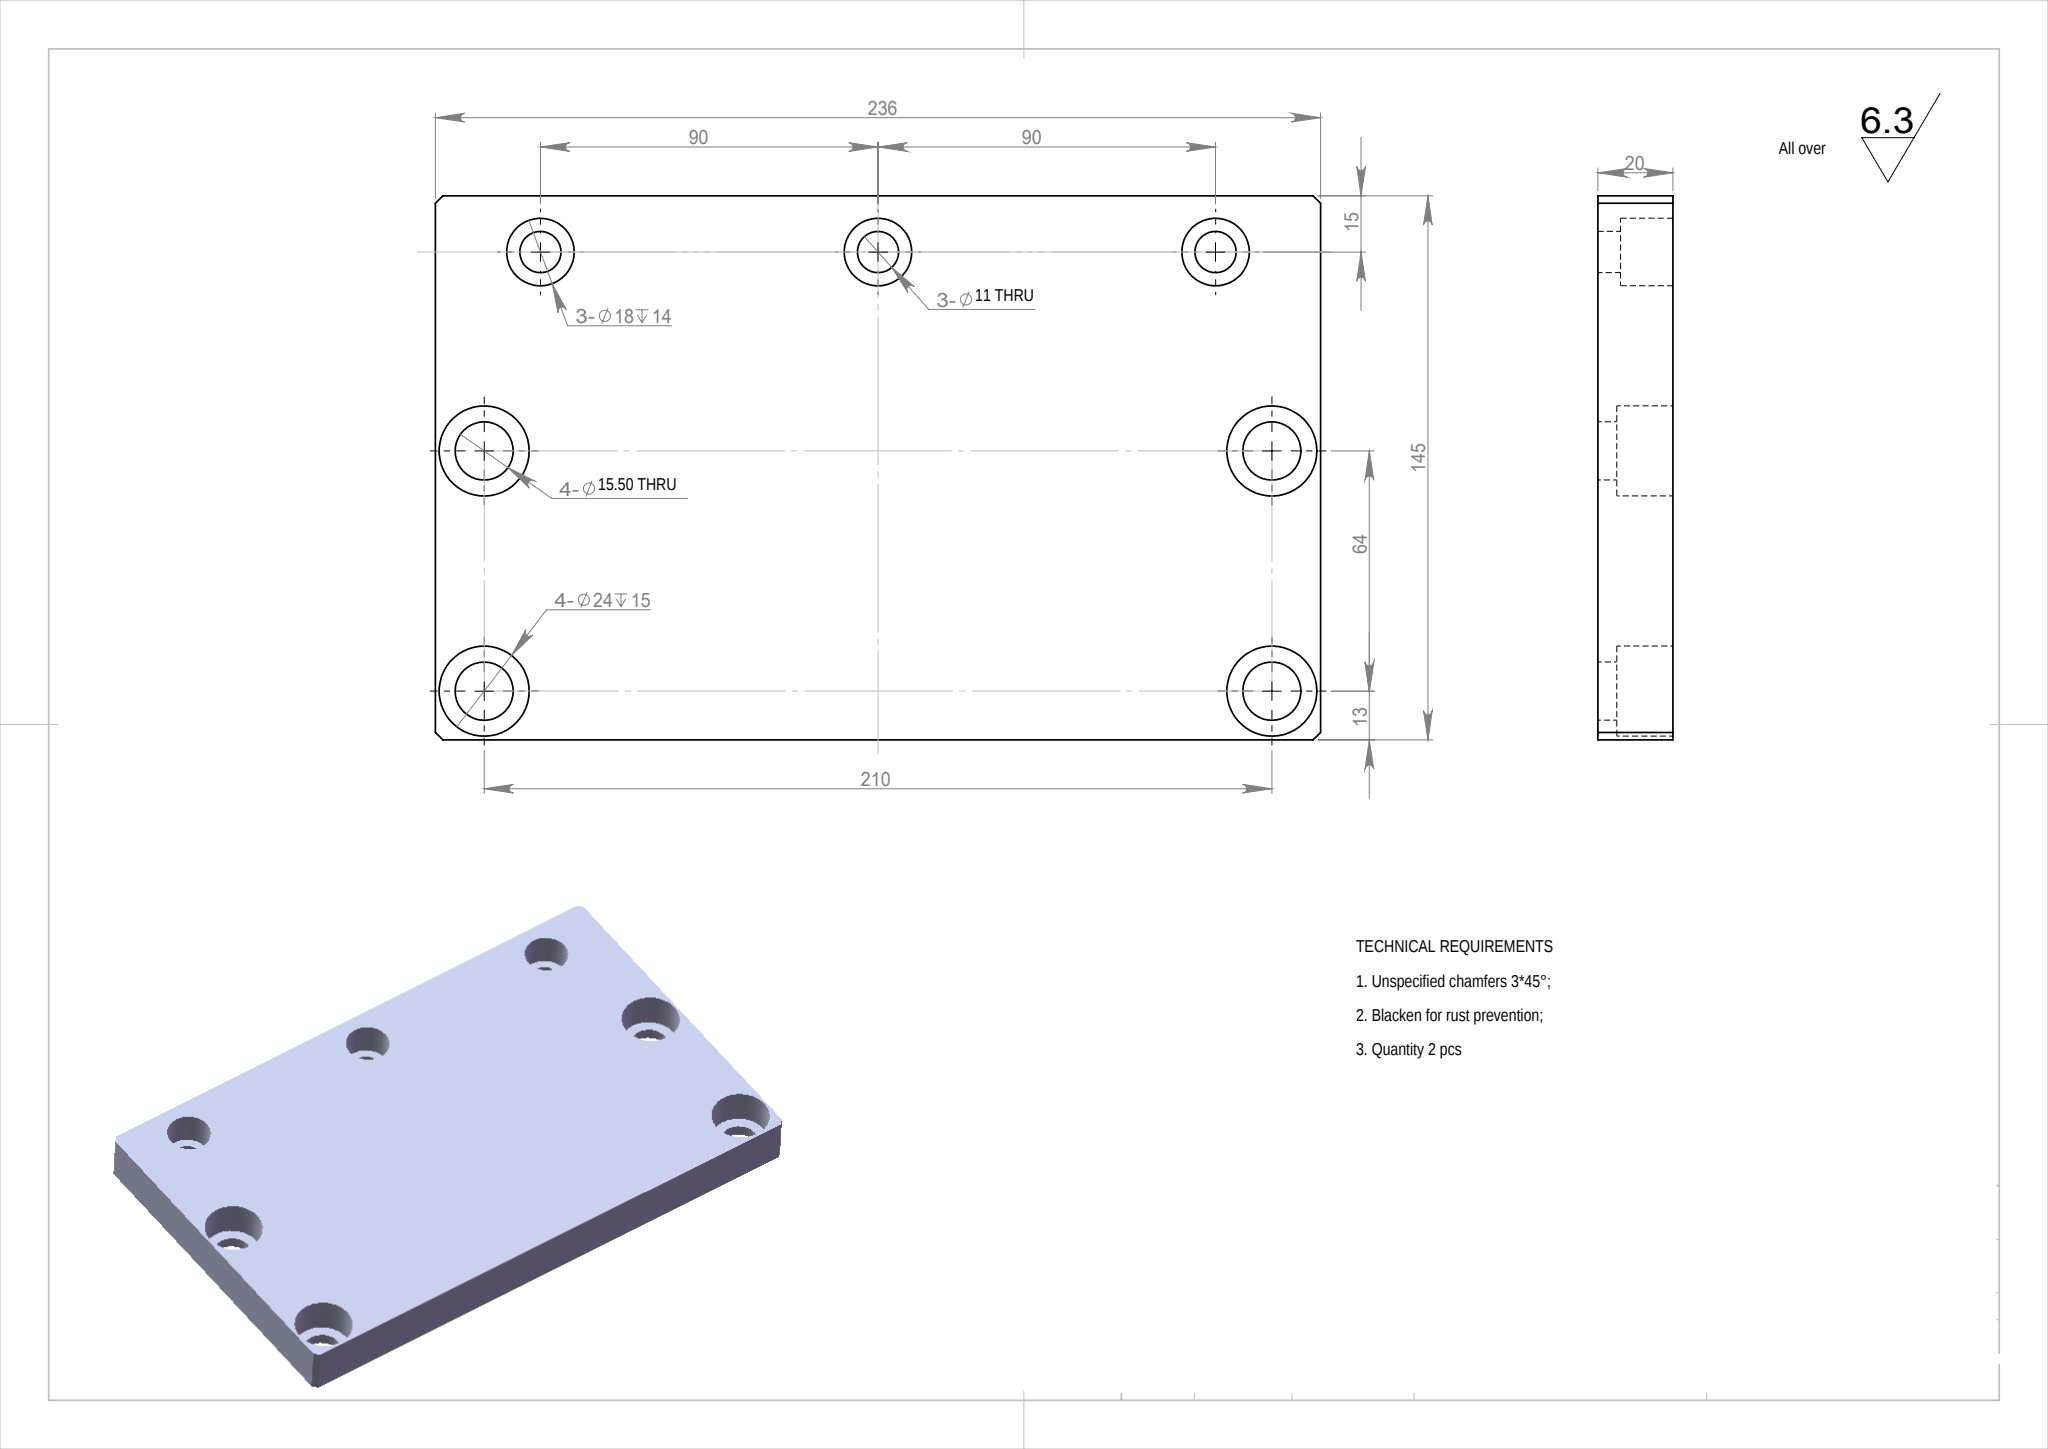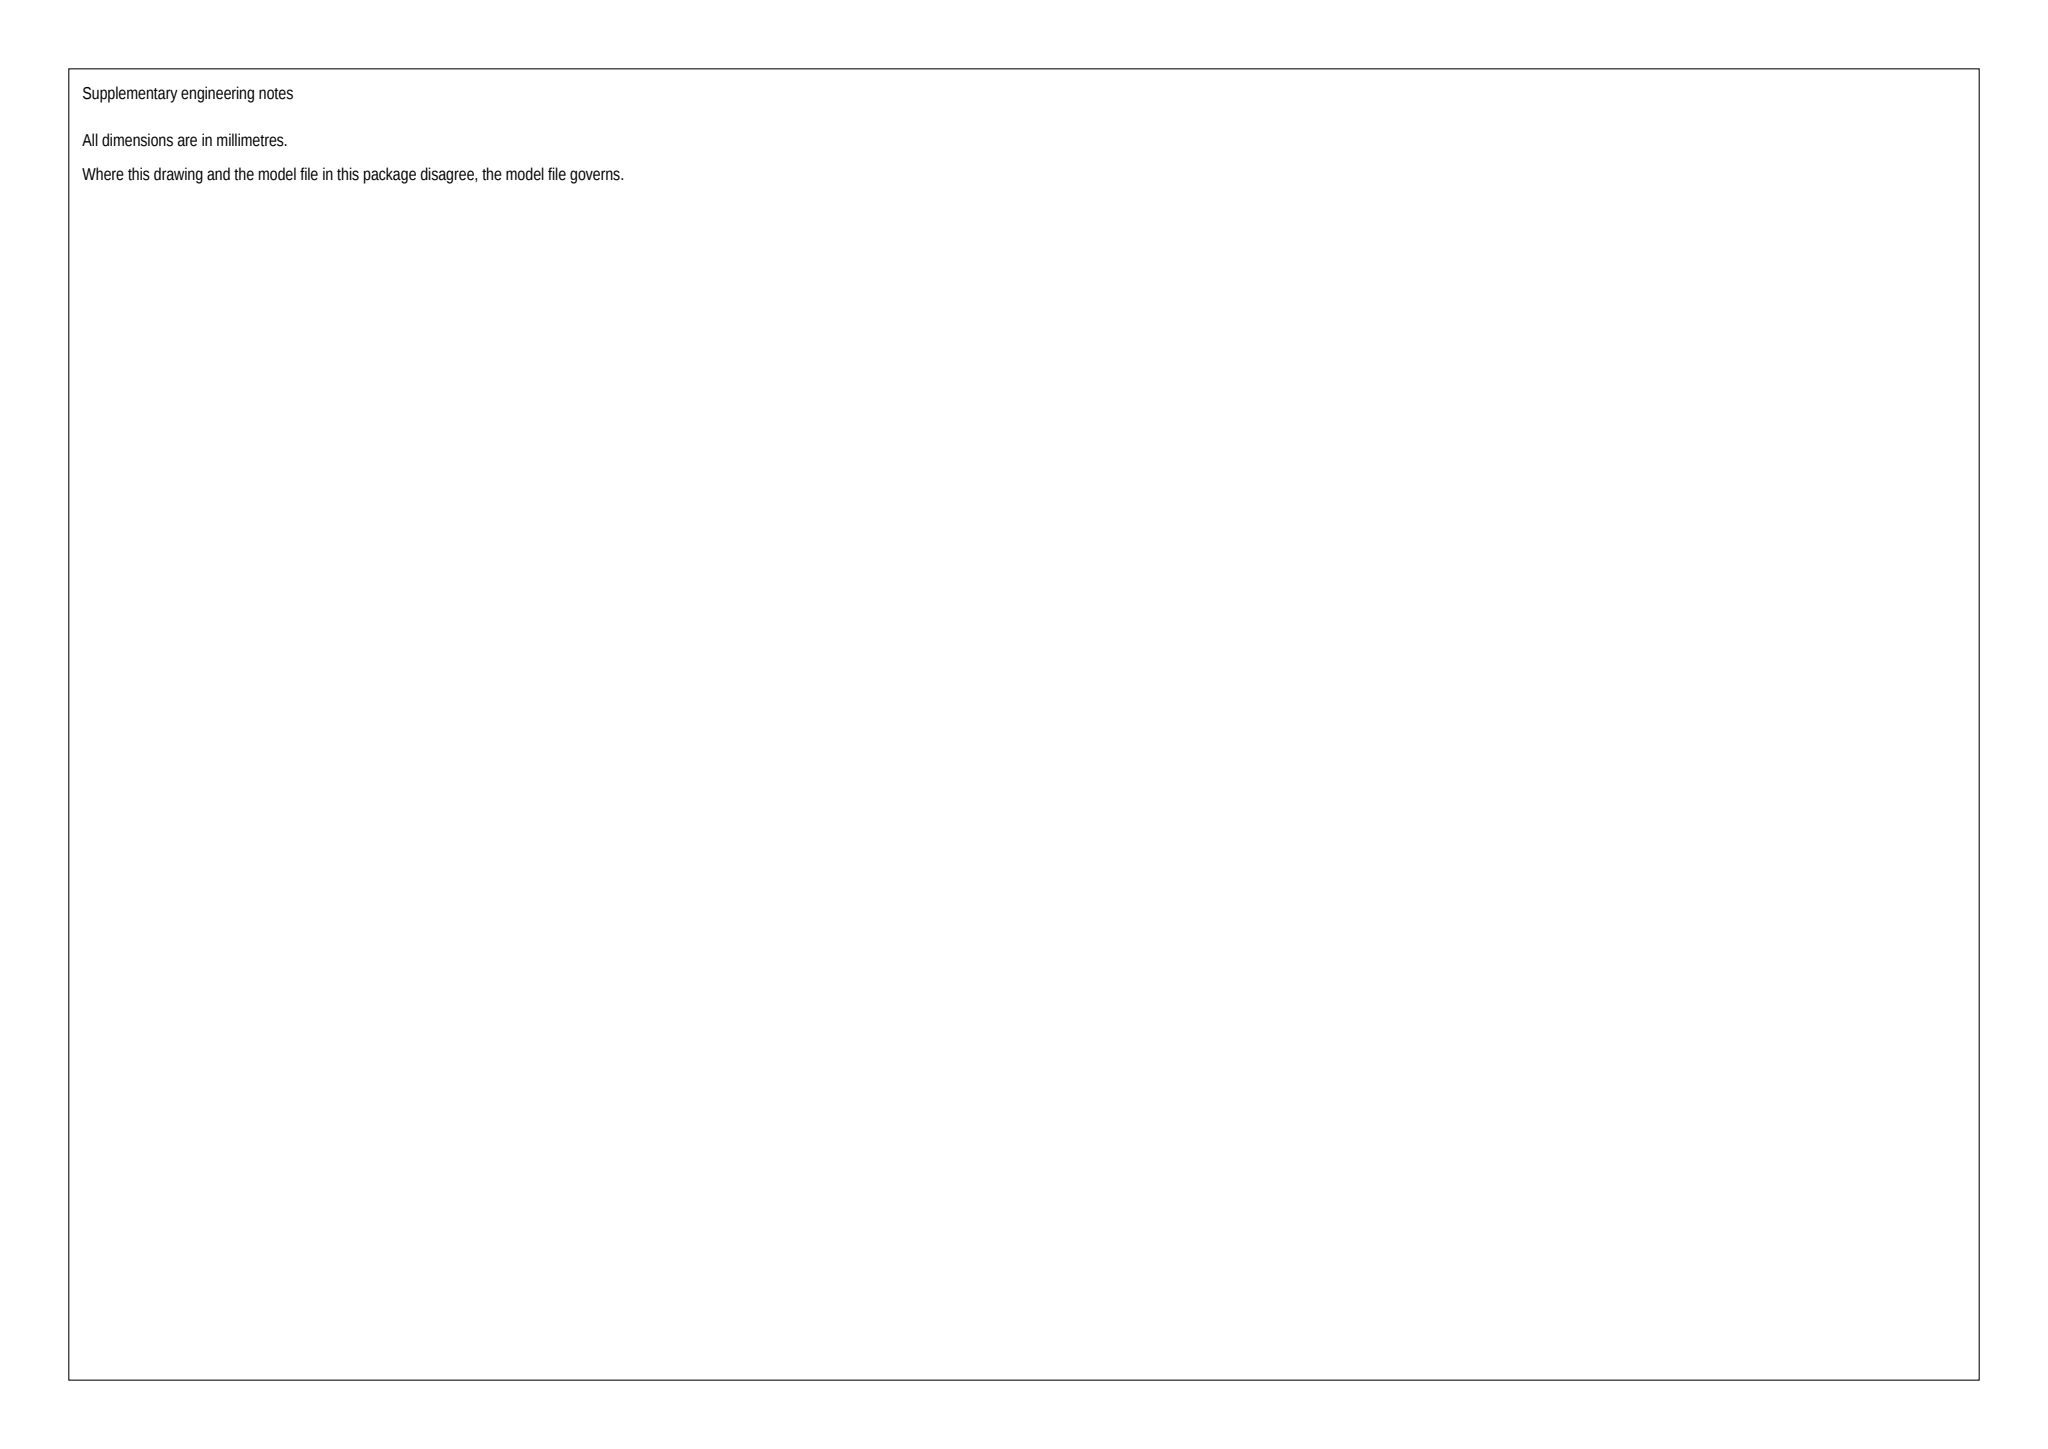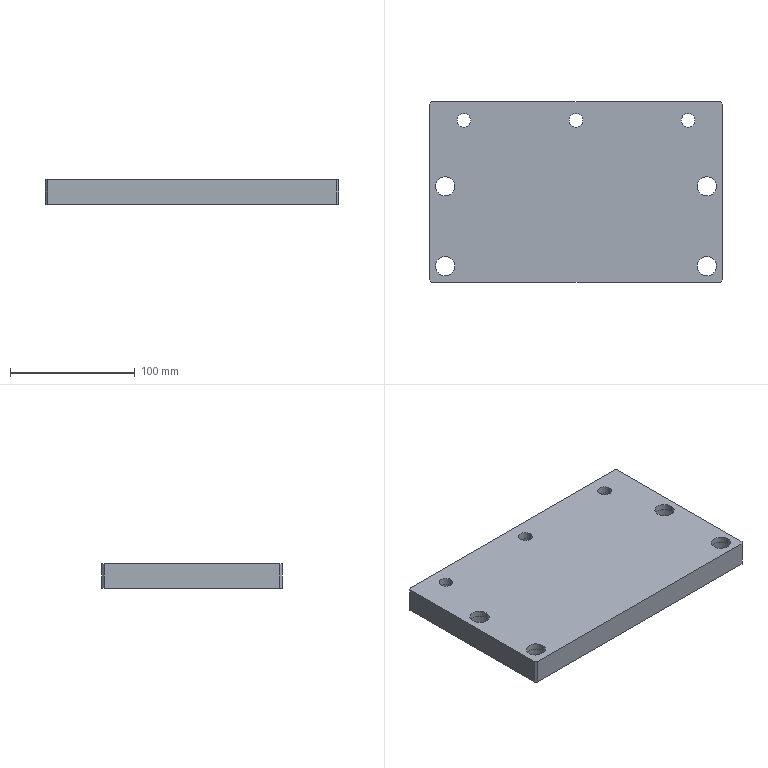Part | SolidWorks | mm | 1 solid | 45 faces | box 236 x 145 x 20 mm | volume 640925 mm3 | cylinder 28 | plane 17 | commonest cylinder face diameters 24 x8 15.5 x8 18 x6 11 x6
Drawing notes:
3-Ø11 / Ø18 DP 14 CL: 28 FROM LEFT EDGE, THEN 90 & 90 | from the solid: Ø11 & Ø18 holes at x=28, 118, 208; bbox x=236
4-Ø15.50 / Ø24 DP 15 CL: 13 FROM EACH SIDE EDGE (210 APART) | from the solid: Ø15.5 & Ø24 holes at x=13 and x=223; bbox x=236
build123d program:
from build123d import *

# Parameters (mm, degrees)
SKETCH1_W                                         = 236
SKETCH1_H                                         = 145
BOSS_EXTRUDE1_DEPTH                               = 20
HOLE_SIZE_ACCORDING_TO_HEXAGON_SOCKET_D           = 15.5
HOLE_SIZE_ACCORDING_TO_HEXAGON_SOCKET_DEPTH       = 24.5
HOLE_SIZE_ACCORDING_TO_HEXAGON_SOCKET_CBORE_D     = 24
HOLE_SIZE_ACCORDING_TO_HEXAGON_SOCKET_CBORE_DEPTH = 15
HOLE_SIZE_ACCORDING_TO_HEXAGON_SOCKET_TIP         = 4.657
HOLE_SIZE_ACCORDING_TO_HEXAGON_SO_2_D             = 11
HOLE_SIZE_ACCORDING_TO_HEXAGON_SO_2_DEPTH         = 24.5
HOLE_SIZE_ACCORDING_TO_HEXAGON_SO_2_CBORE_D       = 18
HOLE_SIZE_ACCORDING_TO_HEXAGON_SO_2_CBORE_DEPTH   = 14
HOLE_SIZE_ACCORDING_TO_HEXAGON_SO_2_TIP           = 3.305
CHAMFER1_SIZE                                     = 2


with BuildPart() as part:
    # Sketch1 → Boss-Extrude1 (new body)
    with BuildSketch(Plane.XY):
        Rectangle(SKETCH1_W, SKETCH1_H)
    extrude(amount=BOSS_EXTRUDE1_DEPTH)

    # Hole Size _ according to_ Hexagon Socket
    with Locations(Plane(origin=(0, 0, 0), x_dir=(-1, 0, 0), z_dir=(0, 0, -1))):
        with Locations((105, 4.5), (105, -59.5), (-105, 4.5), (-105, -59.5)):
            CounterBoreHole(HOLE_SIZE_ACCORDING_TO_HEXAGON_SOCKET_D / 2, HOLE_SIZE_ACCORDING_TO_HEXAGON_SOCKET_CBORE_D / 2, HOLE_SIZE_ACCORDING_TO_HEXAGON_SOCKET_CBORE_DEPTH, depth=HOLE_SIZE_ACCORDING_TO_HEXAGON_SOCKET_DEPTH)
            with Locations((0, 0, -(HOLE_SIZE_ACCORDING_TO_HEXAGON_SOCKET_DEPTH + HOLE_SIZE_ACCORDING_TO_HEXAGON_SOCKET_TIP / 2))):  # 118° drill point
                Cone(0, HOLE_SIZE_ACCORDING_TO_HEXAGON_SOCKET_D / 2, HOLE_SIZE_ACCORDING_TO_HEXAGON_SOCKET_TIP, mode=Mode.SUBTRACT)

    # Hole Size _ according to_ Hexagon So 2
    with Locations(Plane(origin=(0, 0, 0), x_dir=(-1, 0, 0), z_dir=(0, 0, -1))):
        with Locations((90, 57.5), (0, 57.5), (-90, 57.5)):
            CounterBoreHole(HOLE_SIZE_ACCORDING_TO_HEXAGON_SO_2_D / 2, HOLE_SIZE_ACCORDING_TO_HEXAGON_SO_2_CBORE_D / 2, HOLE_SIZE_ACCORDING_TO_HEXAGON_SO_2_CBORE_DEPTH, depth=HOLE_SIZE_ACCORDING_TO_HEXAGON_SO_2_DEPTH)
            with Locations((0, 0, -(HOLE_SIZE_ACCORDING_TO_HEXAGON_SO_2_DEPTH + HOLE_SIZE_ACCORDING_TO_HEXAGON_SO_2_TIP / 2))):  # 118° drill point
                Cone(0, HOLE_SIZE_ACCORDING_TO_HEXAGON_SO_2_D / 2, HOLE_SIZE_ACCORDING_TO_HEXAGON_SO_2_TIP, mode=Mode.SUBTRACT)

    # Chamfer1
    chamfer1_edges = [part.edges().sort_by_distance(p)[0] for p in [
        (118, -72.5, 10),
        (-118, -72.5, 10),
        (-118, 72.5, 10),
        (118, 72.5, 10),
    ]]
    chamfer(chamfer1_edges, length=CHAMFER1_SIZE)


solid = part.part